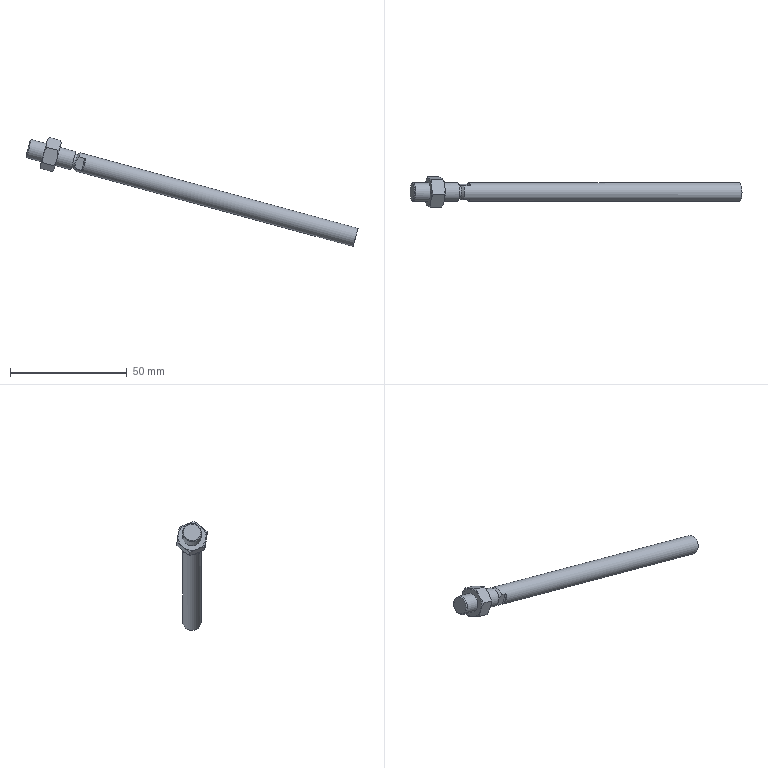Component | NX | HMAC_HS | 2 solids | 36 faces | volume 7672 mm3 | plane 15 | cone 15 | cylinder 6 | commonest cylinder face diameters 8 x3 1 x2 6 x1